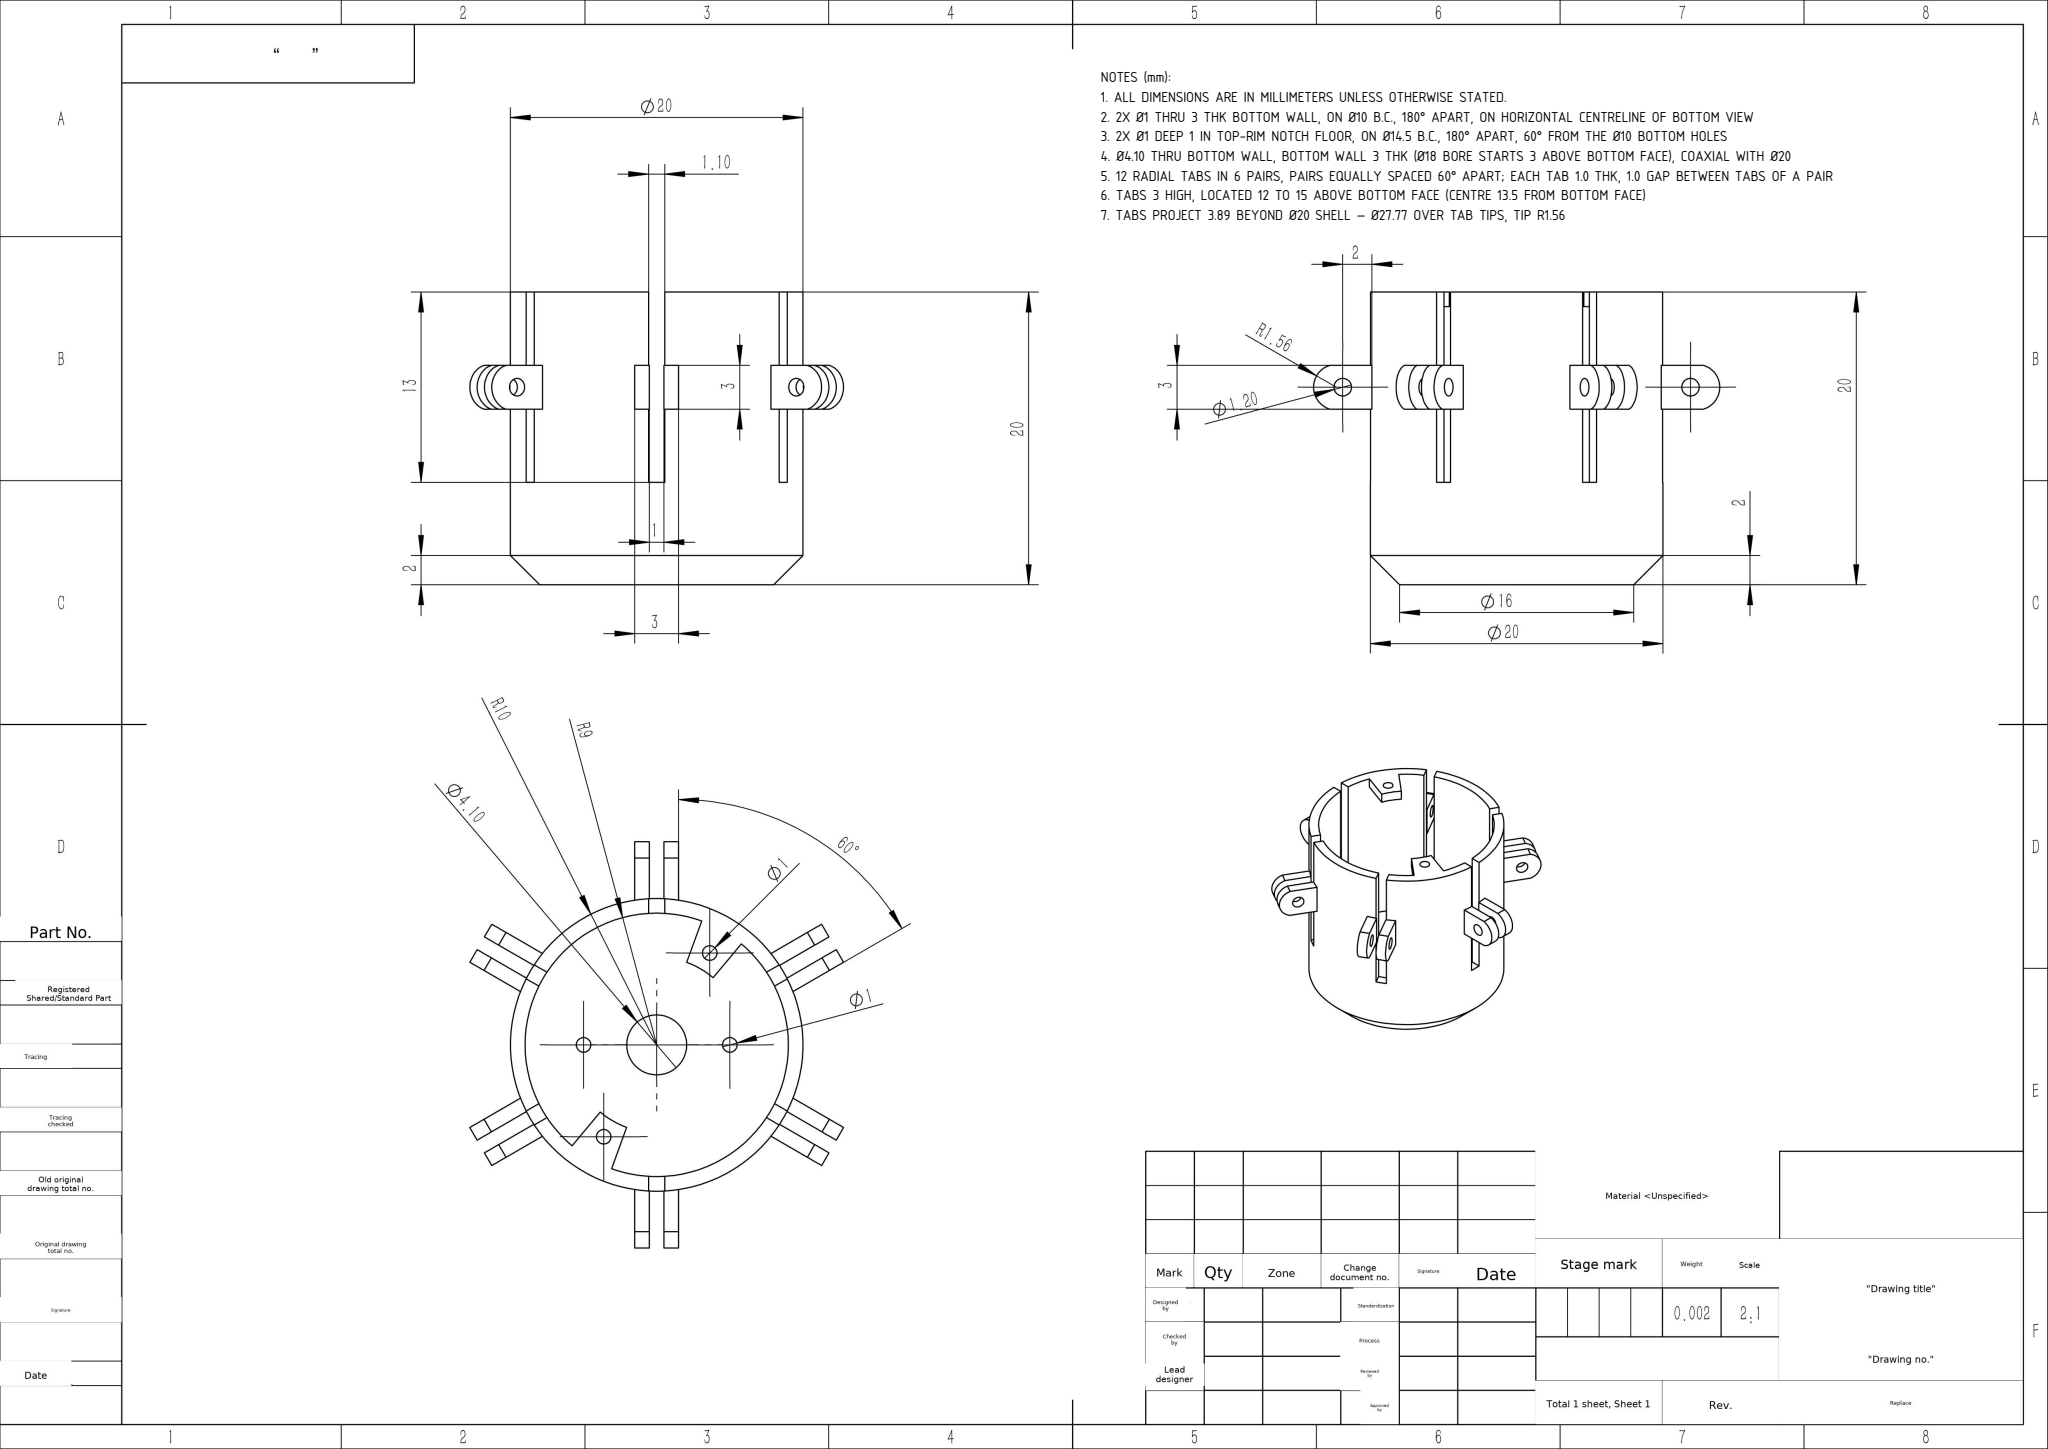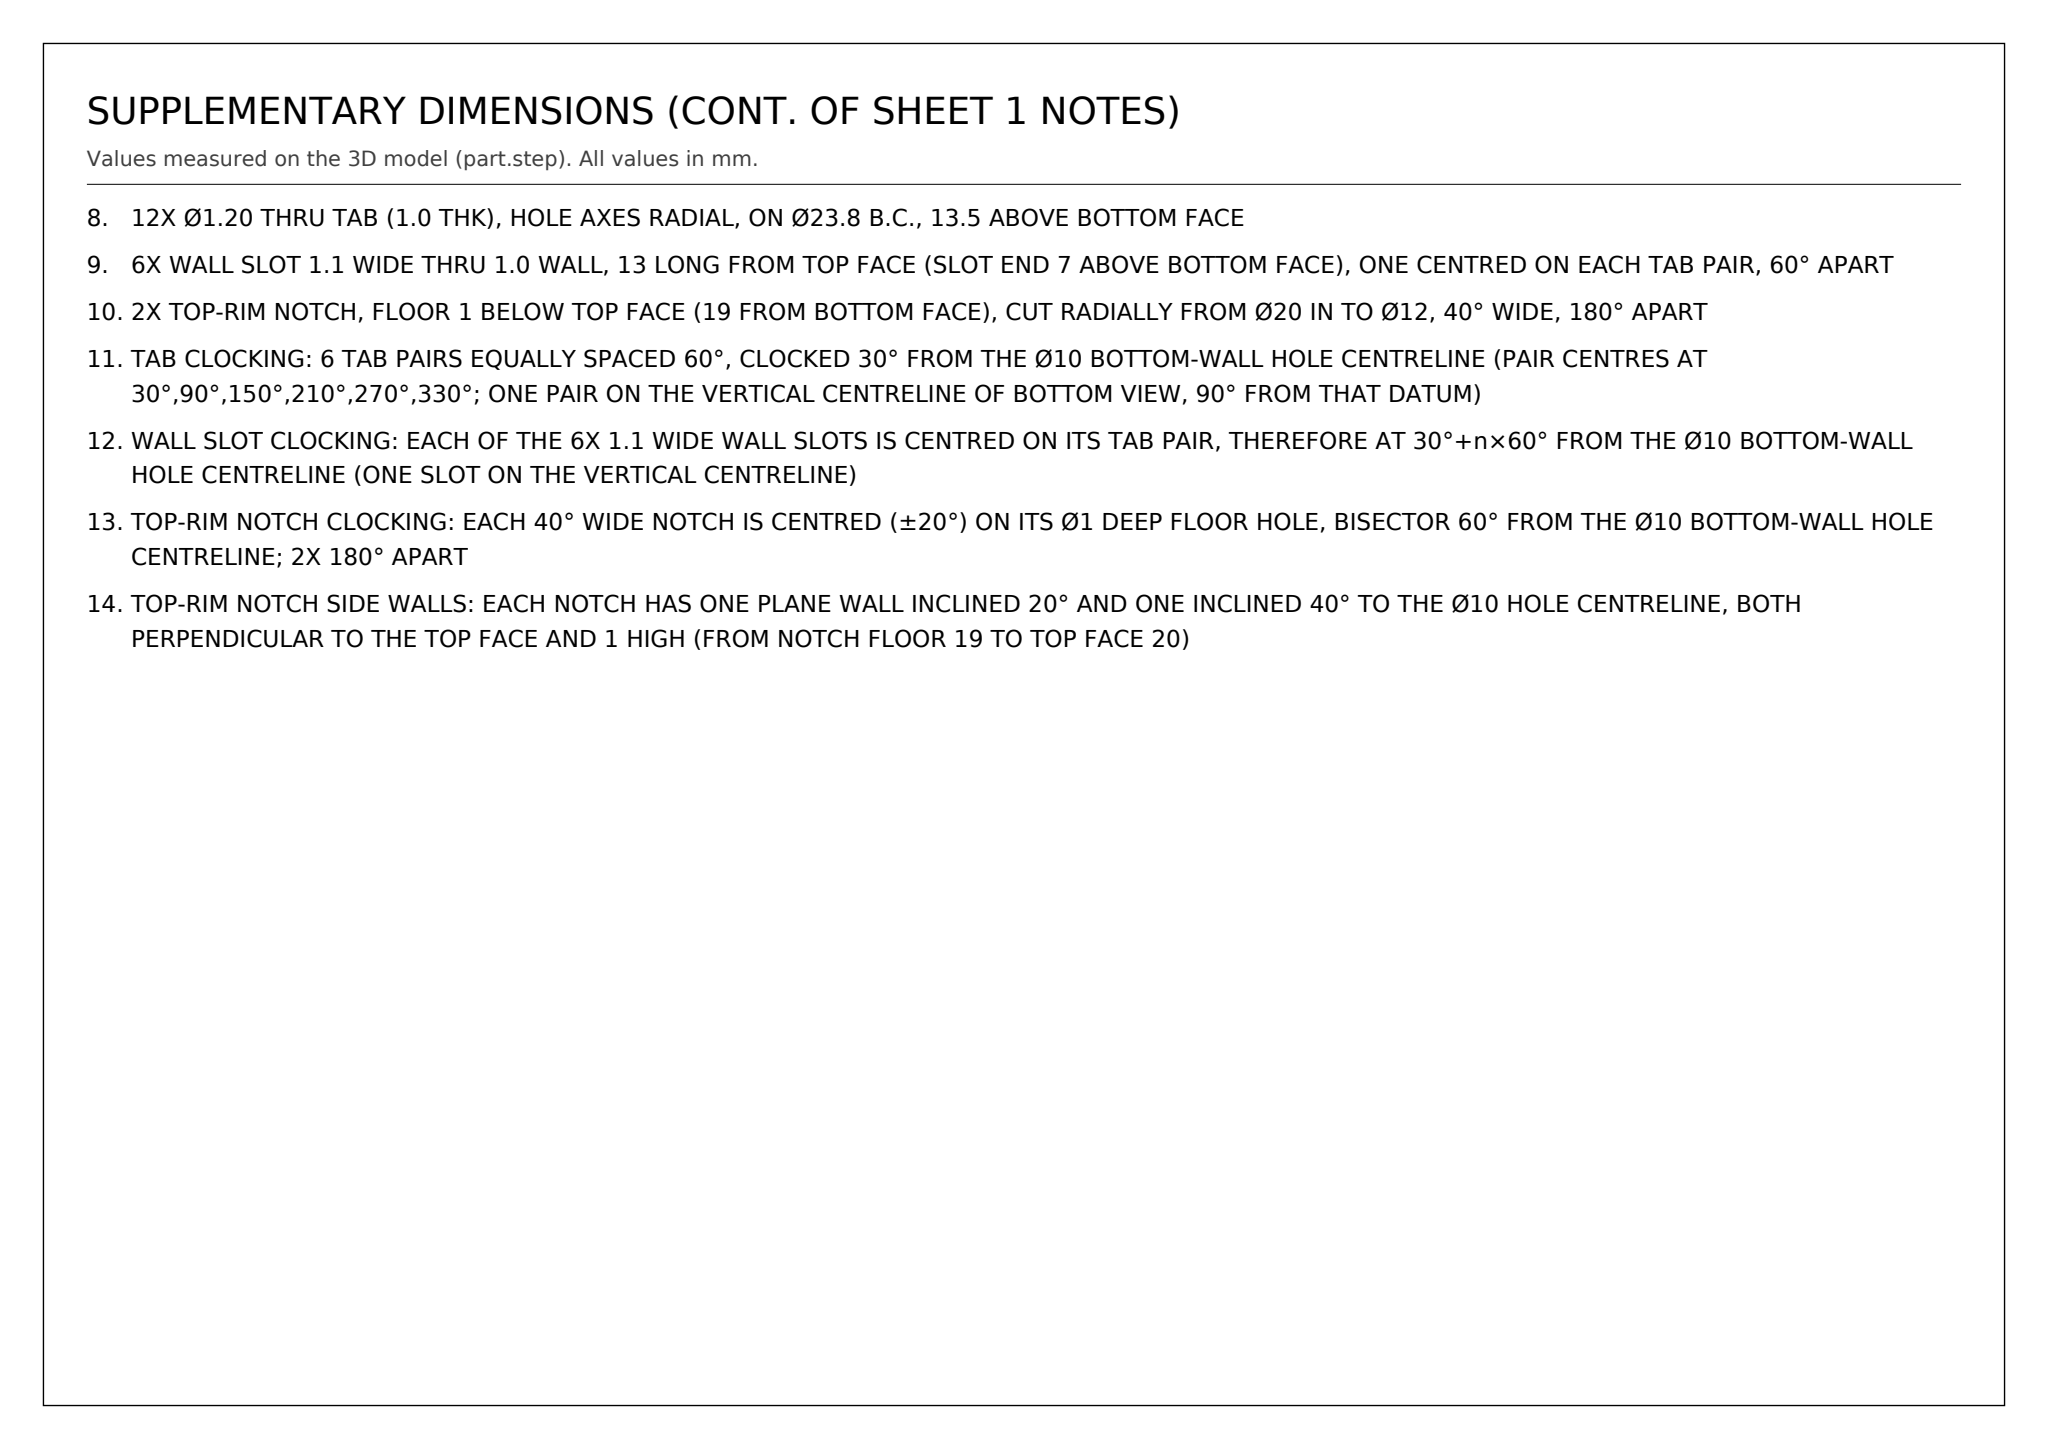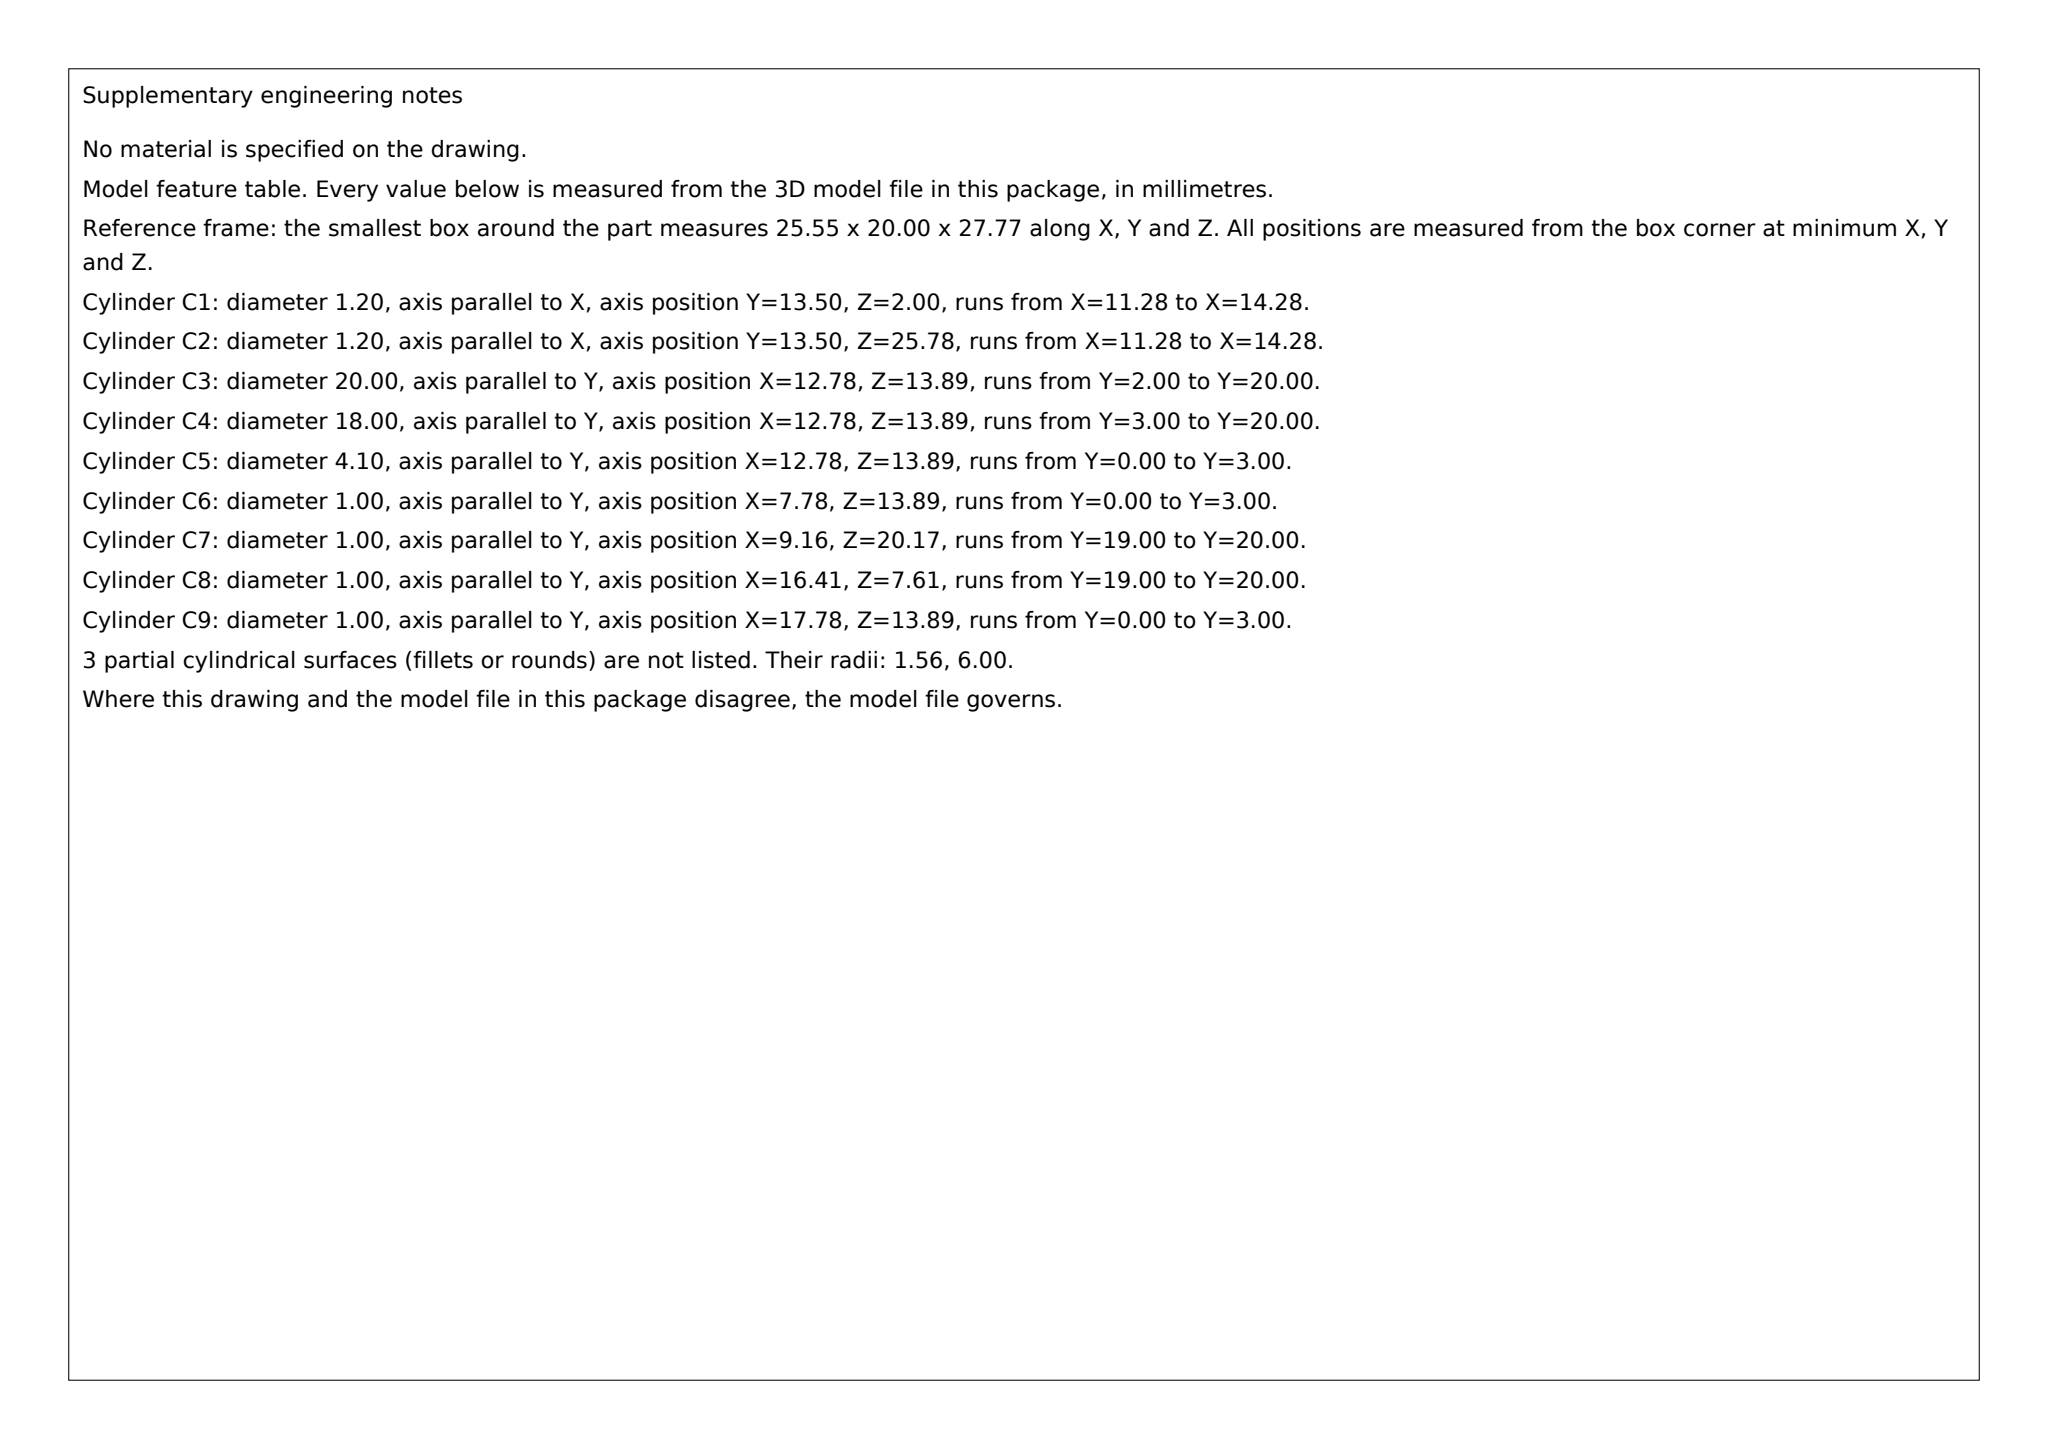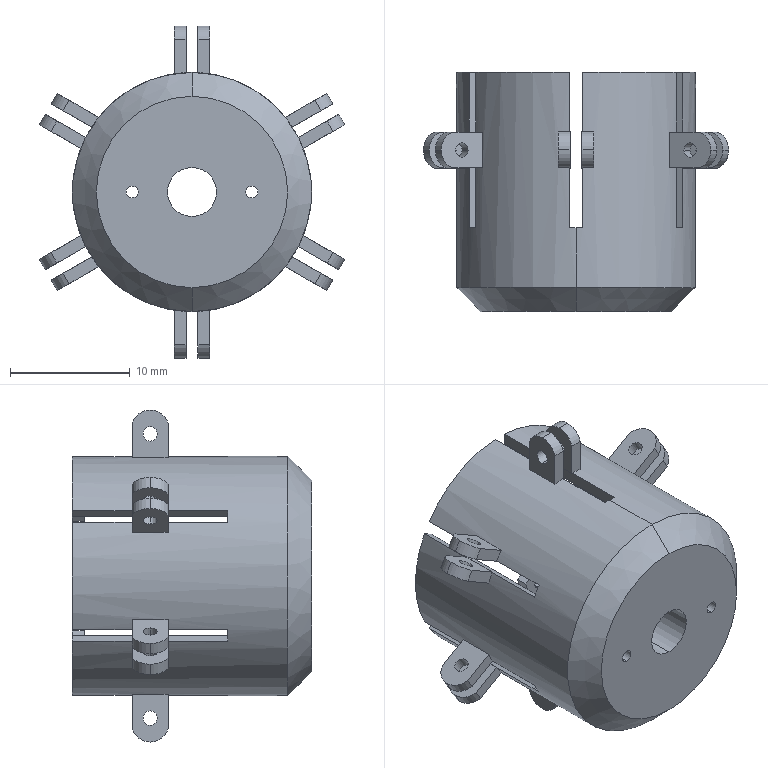Part | SolidWorks | mm | 1 solid | 158 faces | box 25.55 x 20 x 27.77 mm | volume 1842 mm3 | plane 80 | cylinder 76 | cone 2 | commonest cylinder face diameters 1.2 x24 3.125 x24 20 x14 1 x8 4.1 x2 18 x2 12 x2
Drawing notes:
ALL DIMENSIONS ARE IN MILLIMETERS UNLESS OTHERWISE STATED. | from the solid: n/a - sheet-level unit declaration; no STEP dimension value used
2X Ø1 THRU 3 THK BOTTOM WALL, ON Ø10 B.C., 180° APART, ON HORIZONTAL CENTRELINE OF BOTTOM VIEW | from the solid: cylinders: hole/bore Ø1.0 axis y at (7.8,-,13.9) and (17.8,-,13.9), y 0->3; Ø20 shell axis at (12.8,-,13.9) => r=5.0
2X Ø1 DEEP 1 IN TOP-RIM NOTCH FLOOR, ON Ø14.5 B.C., 180° APART, 60° FROM THE Ø10 BOTTOM HOLES | from the solid: cylinders: hole/bore Ø1.0 axis y at (16.4,-,7.6) and (9.2,-,20.2), y 19->20; axis at (12.8,13.9) => r=7.26, 60.3°
Ø4.10 THRU BOTTOM WALL, BOTTOM WALL 3 THK (Ø18 BORE STARTS 3 ABOVE BOTTOM FACE), COAXIAL WITH Ø20 | from the solid: cylinders: hole/bore Ø4.1 axis y at (12.8,-,13.9) y 0->3; hole/bore Ø18 axis y y 3->20
12 RADIAL TABS IN 6 PAIRS, PAIRS EQUALLY SPACED 60° APART; EACH TAB 1.0 THK, 1.0 GAP BETWEEN TABS OF A PAIR | from the solid: axis_planes y=12 / y=15: 12 faces of 3 mm2, e.g. x 11.3-12.3 and x 13.3-14.3 at z 1.1-4.0, repeated at 6 angular locations
TABS 3 HIGH, LOCATED 12 TO 15 ABOVE BOTTOM FACE (CENTRE 13.5 FROM BOTTOM FACE) | from the solid: axis_planes normal y at offsets 12.0 and 15.0 bounding the tab faces; Ø1.20 hole axes at y=13.5
TABS PROJECT 3.89 BEYOND Ø20 SHELL — Ø27.77 OVER TAB TIPS, TIP R1.56 | from the solid: bbox_xyz z = 27.774 vs Ø20 shell axis z=13.9; convex arc Ø3.12 (R1.56) at (-,13.5,1.6)
12X Ø1.20 THRU TAB (1.0 THK), HOLE AXES RADIAL, ON Ø23.8 B.C., 13.5 ABOVE BOTTOM FACE | from the solid: cylinders: hole/bore Ø1.2 axis x at (-,13.5,2.0) and (-,13.5,25.8), x 11.3-12.3 / 13.3-14.3; r = 13.9-2.0 = 11.9
6X WALL SLOT 1.1 WIDE THRU 1.0 WALL, 13 LONG FROM TOP FACE (SLOT END 7 ABOVE BOTTOM FACE), ONE CENTRED ON EACH TAB PAIR, 60° APART | from the solid: axis_planes x=12.2 and x=13.3, extent y 7.0-20.0, z 3.9-4.9 and 22.9-23.9 (wall Ø20/Ø18); inclined planes size (0.9,13.0,0.5) from y=7
2X TOP-RIM NOTCH, FLOOR 1 BELOW TOP FACE (19 FROM BOTTOM FACE), CUT RADIALLY FROM Ø20 IN TO Ø12, 40° WIDE, 180° APART | from the solid: axis_planes y=19.0 extents (14.8-18.6, 5.4-9.3) and (7.0-10.7, 18.5-22.3); concave arc Ø12 axis y at (12.8,-,13.9) y 19->20 arc 40°
TAB CLOCKING: 6 TAB PAIRS EQUALLY SPACED 60°, CLOCKED 30° FROM THE Ø10 BOTTOM-WALL HOLE CENTRELINE (PAIR CENTRES AT 30°,90°,150°,210°,270°,330°; ONE PAIR ON THE VERTICAL CENTRELINE OF BOTTOM VIEW, 90° FROM THAT DATUM) | from the solid: Ø1.2 tab holes with axis along x at [null,13.5,2.0] and [null,13.5,25.8] (z = 13.9 ± 11.9, i.e. on vertical centreline of Ø20 axis at x12.8/z13.9), vs Ø1 bottom-wall holes at [7.8,-,13.9] and [17.8,-,13.9] (on x centreline)
WALL SLOT CLOCKING: EACH OF THE 6X 1.1 WIDE WALL SLOTS IS CENTRED ON ITS TAB PAIR, THEREFORE AT 30°+n×60° FROM THE Ø10 BOTTOM-WALL HOLE CENTRELINE (ONE SLOT ON THE VERTICAL CENTRELINE) | from the solid: slot side faces: planes normal x at 12.2 and 13.3, extent y[7,20] z[3.9,4.9] and z[22.9,23.9] — slot mid-plane x12.75 = Ø20 axis x12.8
TOP-RIM NOTCH CLOCKING: EACH 40° WIDE NOTCH IS CENTRED (±20°) ON ITS Ø1 DEEP FLOOR HOLE, BISECTOR 60° FROM THE Ø10 BOTTOM-WALL HOLE CENTRELINE; 2X 180° APART | from the solid: notch floor planes y=19.0 extent x[14.8,18.6] z[5.4,9.3] and x[7.0,10.7] z[18.5,22.3] centred on Ø1 holes y19-20 at [16.4,-,7.6] and [9.2,-,20.2]; these lie at atan2(±6.3,±3.6)=60° from axis x12.8/z13.9
TOP-RIM NOTCH SIDE WALLS: EACH NOTCH HAS ONE PLANE WALL INCLINED 20° AND ONE INCLINED 40° TO THE Ø10 HOLE CENTRELINE, BOTH PERPENDICULAR TO THE TOP FACE AND 1 HIGH (FROM NOTCH FLOOR 19 TO TOP FACE 20) | from the solid: inclined planes angle_to_xyz [20,90,70] at bbox_from [14.8,19,5.4] and [9.7,19,19.5]; [40,90,50] at bbox_from [16.6,19,7.0] and [7.0,19,18.5], each y-size 1.0